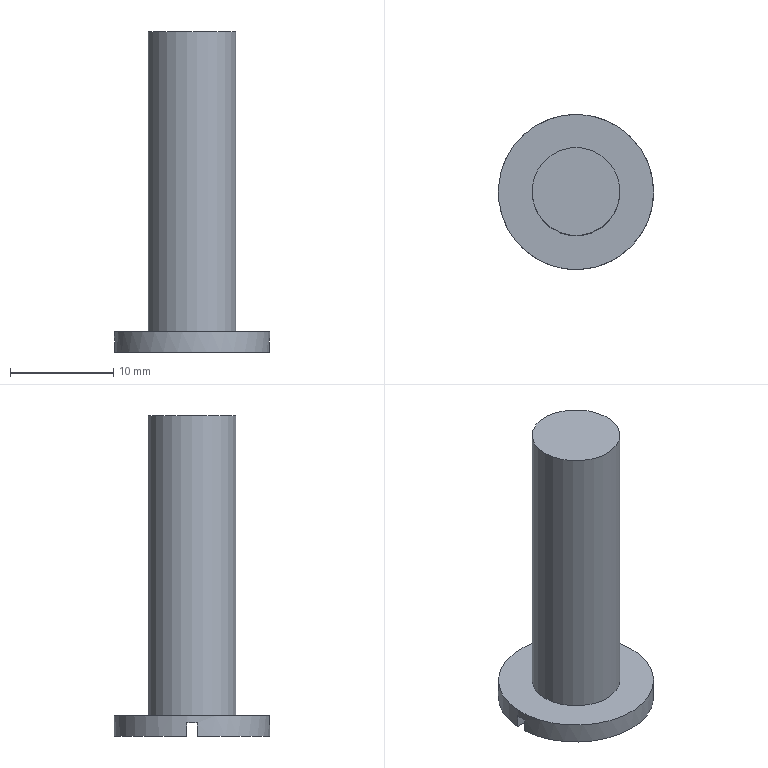Component | NX | ZYD_3 | 1 solid | 9 faces | box 15 x 15 x 31 mm | volume 1980 mm3 | plane 7 | cylinder 2 | commonest cylinder face diameters 15 x1 8.5 x1
STEP:
#1=CARTESIAN_POINT('',(0.,0.,0.));
#2=DIRECTION('',(0.,0.,1.));
#3=DIRECTION('',(1.,0.,0.));
#4=AXIS2_PLACEMENT_3D('',#1,#2,#3);
#5=CARTESIAN_POINT('',(-50.483,0.4989,325.));
#6=VERTEX_POINT('',#5);
#7=CARTESIAN_POINT('',(-35.517,0.4989,325.));
#8=VERTEX_POINT('',#7);
#9=CARTESIAN_POINT('',(-35.517,0.4989,325.));
#10=DIRECTION('',(1.,0.,0.));
#11=VECTOR('',#10,1.);
#12=LINE('',#9,#11);
#13=CARTESIAN_POINT('',(-43.,0.,325.));
#14=DIRECTION('',(0.,0.,1.));
#15=DIRECTION('',(1.,0.,0.));
#16=AXIS2_PLACEMENT_3D('',#13,#14,#15);
#17=PLANE('',#16);
#18=CARTESIAN_POINT('',(7.483,0.4989));
#19=DIRECTION('',(1.,0.));
#20=VECTOR('',#19,1.);
#21=LINE('',#18,#20);
#22=(GEOMETRIC_REPRESENTATION_CONTEXT(2)PARAMETRIC_REPRESENTATION_CONTEXT()REPRESENTATION_CONTEXT('',''));
#23=DEFINITIONAL_REPRESENTATION('',(#21),#22);
#24=PCURVE('',#17,#23);
#25=CARTESIAN_POINT('',(-35.517,0.4989,326.3));
#26=DIRECTION('',(-0.,1.,0.));
#27=DIRECTION('',(-1.,-0.,0.));
#28=AXIS2_PLACEMENT_3D('',#25,#26,#27);
#29=PLANE('',#28);
#30=CARTESIAN_POINT('',(0.,-1.3));
#31=DIRECTION('',(-1.,0.));
#32=VECTOR('',#31,1.);
#33=LINE('',#30,#32);
#34=(GEOMETRIC_REPRESENTATION_CONTEXT(2)PARAMETRIC_REPRESENTATION_CONTEXT()REPRESENTATION_CONTEXT('',''));
#35=DEFINITIONAL_REPRESENTATION('',(#33),#34);
#36=PCURVE('',#29,#35);
#37=SURFACE_CURVE('',#12,(#24,#36),.PCURVE_S1.);
#38=EDGE_CURVE('',#6,#8,#37,.T.);
#39=ORIENTED_EDGE('',*,*,#38,.F.);
#40=CARTESIAN_POINT('',(-43.,0.,325.));
#41=DIRECTION('',(0.,0.,1.));
#42=DIRECTION('',(1.,0.,0.));
#43=AXIS2_PLACEMENT_3D('',#40,#41,#42);
#44=CIRCLE('',#43,7.5);
#45=CARTESIAN_POINT('',(0.,0.));
#46=DIRECTION('',(1.,0.));
#47=AXIS2_PLACEMENT_2D('',#45,#46);
#48=CIRCLE('',#47,7.5);
#49=(GEOMETRIC_REPRESENTATION_CONTEXT(2)PARAMETRIC_REPRESENTATION_CONTEXT()REPRESENTATION_CONTEXT('',''));
#50=DEFINITIONAL_REPRESENTATION('',(#48),#49);
#51=PCURVE('',#17,#50);
#52=CARTESIAN_POINT('',(-43.,0.,327.));
#53=DIRECTION('',(0.,0.,-1.));
#54=DIRECTION('',(-1.,0.,0.));
#55=AXIS2_PLACEMENT_3D('',#52,#53,#54);
#56=CYLINDRICAL_SURFACE('',#55,7.5);
#57=CARTESIAN_POINT('',(3.142,2.));
#58=DIRECTION('',(-1.,0.));
#59=VECTOR('',#58,1.);
#60=LINE('',#57,#59);
#61=(GEOMETRIC_REPRESENTATION_CONTEXT(2)PARAMETRIC_REPRESENTATION_CONTEXT()REPRESENTATION_CONTEXT('',''));
#62=DEFINITIONAL_REPRESENTATION('',(#60),#61);
#63=PCURVE('',#56,#62);
#64=SURFACE_CURVE('',#44,(#51,#63),.PCURVE_S1.);
#65=EDGE_CURVE('',#8,#6,#64,.T.);
#66=ORIENTED_EDGE('',*,*,#65,.F.);
#67=EDGE_LOOP('',(#39,#66));
#68=FACE_BOUND('',#67,.T.);
#69=ADVANCED_FACE('',(#68),#17,.F.);
#70=CARTESIAN_POINT('',(-35.517,-0.4989,325.));
#71=VERTEX_POINT('',#70);
#72=CARTESIAN_POINT('',(-50.483,-0.4989,325.));
#73=VERTEX_POINT('',#72);
#74=CARTESIAN_POINT('',(-50.483,-0.4989,325.));
#75=DIRECTION('',(-1.,0.,0.));
#76=VECTOR('',#75,1.);
#77=LINE('',#74,#76);
#78=CARTESIAN_POINT('',(-43.,0.,325.));
#79=DIRECTION('',(0.,0.,1.));
#80=DIRECTION('',(1.,0.,0.));
#81=AXIS2_PLACEMENT_3D('',#78,#79,#80);
#82=PLANE('',#81);
#83=CARTESIAN_POINT('',(-7.483,-0.4989));
#84=DIRECTION('',(-1.,0.));
#85=VECTOR('',#84,1.);
#86=LINE('',#83,#85);
#87=(GEOMETRIC_REPRESENTATION_CONTEXT(2)PARAMETRIC_REPRESENTATION_CONTEXT()REPRESENTATION_CONTEXT('',''));
#88=DEFINITIONAL_REPRESENTATION('',(#86),#87);
#89=PCURVE('',#82,#88);
#90=CARTESIAN_POINT('',(-50.483,-0.4989,326.3));
#91=DIRECTION('',(0.,-1.,0.));
#92=DIRECTION('',(0.,0.,-1.));
#93=AXIS2_PLACEMENT_3D('',#90,#91,#92);
#94=PLANE('',#93);
#95=CARTESIAN_POINT('',(1.3,0.));
#96=DIRECTION('',(0.,-1.));
#97=VECTOR('',#96,1.);
#98=LINE('',#95,#97);
#99=(GEOMETRIC_REPRESENTATION_CONTEXT(2)PARAMETRIC_REPRESENTATION_CONTEXT()REPRESENTATION_CONTEXT('',''));
#100=DEFINITIONAL_REPRESENTATION('',(#98),#99);
#101=PCURVE('',#94,#100);
#102=SURFACE_CURVE('',#77,(#89,#101),.PCURVE_S1.);
#103=EDGE_CURVE('',#71,#73,#102,.T.);
#104=ORIENTED_EDGE('',*,*,#103,.F.);
#105=CARTESIAN_POINT('',(-43.,0.,325.));
#106=DIRECTION('',(0.,0.,1.));
#107=DIRECTION('',(1.,0.,0.));
#108=AXIS2_PLACEMENT_3D('',#105,#106,#107);
#109=CIRCLE('',#108,7.5);
#110=CARTESIAN_POINT('',(0.,0.));
#111=DIRECTION('',(1.,0.));
#112=AXIS2_PLACEMENT_2D('',#110,#111);
#113=CIRCLE('',#112,7.5);
#114=(GEOMETRIC_REPRESENTATION_CONTEXT(2)PARAMETRIC_REPRESENTATION_CONTEXT()REPRESENTATION_CONTEXT('',''));
#115=DEFINITIONAL_REPRESENTATION('',(#113),#114);
#116=PCURVE('',#82,#115);
#117=CARTESIAN_POINT('',(9.425,2.));
#118=DIRECTION('',(-1.,0.));
#119=VECTOR('',#118,1.);
#120=LINE('',#117,#119);
#121=(GEOMETRIC_REPRESENTATION_CONTEXT(2)PARAMETRIC_REPRESENTATION_CONTEXT()REPRESENTATION_CONTEXT('',''));
#122=DEFINITIONAL_REPRESENTATION('',(#120),#121);
#123=PCURVE('',#56,#122);
#124=SURFACE_CURVE('',#109,(#116,#123),.PCURVE_S1.);
#125=EDGE_CURVE('',#73,#71,#124,.T.);
#126=ORIENTED_EDGE('',*,*,#125,.F.);
#127=EDGE_LOOP('',(#104,#126));
#128=FACE_BOUND('',#127,.T.);
#129=ADVANCED_FACE('',(#128),#82,.F.);
#130=CARTESIAN_POINT('',(-35.517,0.4989,326.3));
#131=VERTEX_POINT('',#130);
#132=CARTESIAN_POINT('',(-35.517,-0.4989,326.3));
#133=VERTEX_POINT('',#132);
#134=CARTESIAN_POINT('',(-43.,0.,326.3));
#135=DIRECTION('',(0.,0.,-1.));
#136=DIRECTION('',(-1.,0.,0.));
#137=AXIS2_PLACEMENT_3D('',#134,#135,#136);
#138=CIRCLE('',#137,7.5);
#139=CARTESIAN_POINT('',(0.,0.7));
#140=DIRECTION('',(1.,0.));
#141=VECTOR('',#140,1.);
#142=LINE('',#139,#141);
#143=(GEOMETRIC_REPRESENTATION_CONTEXT(2)PARAMETRIC_REPRESENTATION_CONTEXT()REPRESENTATION_CONTEXT('',''));
#144=DEFINITIONAL_REPRESENTATION('',(#142),#143);
#145=PCURVE('',#56,#144);
#146=CARTESIAN_POINT('',(-52.183,0.4989,326.3));
#147=DIRECTION('',(0.,0.,-1.));
#148=DIRECTION('',(-1.,0.,0.));
#149=AXIS2_PLACEMENT_3D('',#146,#147,#148);
#150=PLANE('',#149);
#151=CARTESIAN_POINT('',(-9.183,-0.4989));
#152=DIRECTION('',(1.,0.));
#153=AXIS2_PLACEMENT_2D('',#151,#152);
#154=CIRCLE('',#153,7.5);
#155=(GEOMETRIC_REPRESENTATION_CONTEXT(2)PARAMETRIC_REPRESENTATION_CONTEXT()REPRESENTATION_CONTEXT('',''));
#156=DEFINITIONAL_REPRESENTATION('',(#154),#155);
#157=PCURVE('',#150,#156);
#158=SURFACE_CURVE('',#138,(#145,#157),.PCURVE_S1.);
#159=EDGE_CURVE('',#131,#133,#158,.T.);
#160=ORIENTED_EDGE('',*,*,#159,.F.);
#161=CARTESIAN_POINT('',(-35.517,0.4989,327.));
#162=DIRECTION('',(0.,0.,-1.));
#163=VECTOR('',#162,1.);
#164=LINE('',#161,#163);
#165=CARTESIAN_POINT('',(3.075,0.));
#166=DIRECTION('',(0.,1.));
#167=VECTOR('',#166,1.);
#168=LINE('',#165,#167);
#169=(GEOMETRIC_REPRESENTATION_CONTEXT(2)PARAMETRIC_REPRESENTATION_CONTEXT()REPRESENTATION_CONTEXT('',''));
#170=DEFINITIONAL_REPRESENTATION('',(#168),#169);
#171=PCURVE('',#56,#170);
#172=CARTESIAN_POINT('',(0.,0.7));
#173=DIRECTION('',(0.,-1.));
#174=VECTOR('',#173,1.);
#175=LINE('',#172,#174);
#176=(GEOMETRIC_REPRESENTATION_CONTEXT(2)PARAMETRIC_REPRESENTATION_CONTEXT()REPRESENTATION_CONTEXT('',''));
#177=DEFINITIONAL_REPRESENTATION('',(#175),#176);
#178=PCURVE('',#29,#177);
#179=SURFACE_CURVE('',#164,(#171,#178),.PCURVE_S1.);
#180=EDGE_CURVE('',#131,#8,#179,.T.);
#181=ORIENTED_EDGE('',*,*,#180,.T.);
#182=ORIENTED_EDGE('',*,*,#65,.T.);
#183=CARTESIAN_POINT('',(-50.483,0.4989,326.3));
#184=VERTEX_POINT('',#183);
#185=CARTESIAN_POINT('',(-50.483,0.4989,327.));
#186=DIRECTION('',(0.,0.,1.));
#187=VECTOR('',#186,1.);
#188=LINE('',#185,#187);
#189=CARTESIAN_POINT('',(0.06657,0.));
#190=DIRECTION('',(0.,-1.));
#191=VECTOR('',#190,1.);
#192=LINE('',#189,#191);
#193=(GEOMETRIC_REPRESENTATION_CONTEXT(2)PARAMETRIC_REPRESENTATION_CONTEXT()REPRESENTATION_CONTEXT('',''));
#194=DEFINITIONAL_REPRESENTATION('',(#192),#193);
#195=PCURVE('',#56,#194);
#196=CARTESIAN_POINT('',(14.967,0.7));
#197=DIRECTION('',(0.,1.));
#198=VECTOR('',#197,1.);
#199=LINE('',#196,#198);
#200=(GEOMETRIC_REPRESENTATION_CONTEXT(2)PARAMETRIC_REPRESENTATION_CONTEXT()REPRESENTATION_CONTEXT('',''));
#201=DEFINITIONAL_REPRESENTATION('',(#199),#200);
#202=PCURVE('',#29,#201);
#203=SURFACE_CURVE('',#188,(#195,#202),.PCURVE_S1.);
#204=EDGE_CURVE('',#6,#184,#203,.T.);
#205=ORIENTED_EDGE('',*,*,#204,.T.);
#206=CARTESIAN_POINT('',(-50.483,0.4989,327.));
#207=VERTEX_POINT('',#206);
#208=CARTESIAN_POINT('',(-50.483,0.4989,327.));
#209=CARTESIAN_POINT('',(-50.483,0.4989,326.3));
#210=B_SPLINE_CURVE_WITH_KNOTS('',1,(#208,#209),.UNSPECIFIED.,.F.,.F.,(2,2),(0.,0.7),.PIECEWISE_BEZIER_KNOTS.);
#211=CARTESIAN_POINT('',(0.06657,0.));
#212=DIRECTION('',(0.,1.));
#213=VECTOR('',#212,1.);
#214=LINE('',#211,#213);
#215=(GEOMETRIC_REPRESENTATION_CONTEXT(2)PARAMETRIC_REPRESENTATION_CONTEXT()REPRESENTATION_CONTEXT('',''));
#216=DEFINITIONAL_REPRESENTATION('',(#214),#215);
#217=PCURVE('',#56,#216);
#218=CARTESIAN_POINT('',(6.35,0.));
#219=DIRECTION('',(0.,1.));
#220=VECTOR('',#219,1.);
#221=LINE('',#218,#220);
#222=(GEOMETRIC_REPRESENTATION_CONTEXT(2)PARAMETRIC_REPRESENTATION_CONTEXT()REPRESENTATION_CONTEXT('',''));
#223=DEFINITIONAL_REPRESENTATION('',(#221),#222);
#224=PCURVE('',#56,#223);
#225=SEAM_CURVE('',#210,(#217,#224),.PCURVE_S1.);
#226=EDGE_CURVE('',#207,#184,#225,.T.);
#227=ORIENTED_EDGE('',*,*,#226,.F.);
#228=CARTESIAN_POINT('',(-35.5,0.,327.));
#229=VERTEX_POINT('',#228);
#230=CARTESIAN_POINT('',(-43.,0.,327.));
#231=DIRECTION('',(0.,0.,1.));
#232=DIRECTION('',(1.,0.,0.));
#233=AXIS2_PLACEMENT_3D('',#230,#231,#232);
#234=CIRCLE('',#233,7.5);
#235=CARTESIAN_POINT('',(3.142,0.));
#236=DIRECTION('',(-1.,0.));
#237=VECTOR('',#236,1.);
#238=LINE('',#235,#237);
#239=(GEOMETRIC_REPRESENTATION_CONTEXT(2)PARAMETRIC_REPRESENTATION_CONTEXT()REPRESENTATION_CONTEXT('',''));
#240=DEFINITIONAL_REPRESENTATION('',(#238),#239);
#241=PCURVE('',#56,#240);
#242=CARTESIAN_POINT('',(-43.,0.,327.));
#243=DIRECTION('',(0.,0.,1.));
#244=DIRECTION('',(1.,0.,0.));
#245=AXIS2_PLACEMENT_3D('',#242,#243,#244);
#246=PLANE('',#245);
#247=CARTESIAN_POINT('',(0.,0.));
#248=DIRECTION('',(1.,0.));
#249=AXIS2_PLACEMENT_2D('',#247,#248);
#250=CIRCLE('',#249,7.5);
#251=(GEOMETRIC_REPRESENTATION_CONTEXT(2)PARAMETRIC_REPRESENTATION_CONTEXT()REPRESENTATION_CONTEXT('',''));
#252=DEFINITIONAL_REPRESENTATION('',(#250),#251);
#253=PCURVE('',#246,#252);
#254=SURFACE_CURVE('',#234,(#241,#253),.PCURVE_S1.);
#255=EDGE_CURVE('',#229,#207,#254,.T.);
#256=ORIENTED_EDGE('',*,*,#255,.F.);
#257=CARTESIAN_POINT('',(-43.,0.,327.));
#258=DIRECTION('',(0.,0.,1.));
#259=DIRECTION('',(1.,0.,0.));
#260=AXIS2_PLACEMENT_3D('',#257,#258,#259);
#261=CIRCLE('',#260,7.5);
#262=CARTESIAN_POINT('',(9.425,0.));
#263=DIRECTION('',(-1.,0.));
#264=VECTOR('',#263,1.);
#265=LINE('',#262,#264);
#266=(GEOMETRIC_REPRESENTATION_CONTEXT(2)PARAMETRIC_REPRESENTATION_CONTEXT()REPRESENTATION_CONTEXT('',''));
#267=DEFINITIONAL_REPRESENTATION('',(#265),#266);
#268=PCURVE('',#56,#267);
#269=CARTESIAN_POINT('',(0.,0.));
#270=DIRECTION('',(1.,0.));
#271=AXIS2_PLACEMENT_2D('',#269,#270);
#272=CIRCLE('',#271,7.5);
#273=(GEOMETRIC_REPRESENTATION_CONTEXT(2)PARAMETRIC_REPRESENTATION_CONTEXT()REPRESENTATION_CONTEXT('',''));
#274=DEFINITIONAL_REPRESENTATION('',(#272),#273);
#275=PCURVE('',#246,#274);
#276=SURFACE_CURVE('',#261,(#268,#275),.PCURVE_S1.);
#277=EDGE_CURVE('',#207,#229,#276,.T.);
#278=ORIENTED_EDGE('',*,*,#277,.F.);
#279=ORIENTED_EDGE('',*,*,#226,.T.);
#280=CARTESIAN_POINT('',(-50.483,-0.4989,326.3));
#281=VERTEX_POINT('',#280);
#282=CARTESIAN_POINT('',(-43.,0.,326.3));
#283=DIRECTION('',(0.,0.,-1.));
#284=DIRECTION('',(-1.,0.,0.));
#285=AXIS2_PLACEMENT_3D('',#282,#283,#284);
#286=CIRCLE('',#285,7.5);
#287=CARTESIAN_POINT('',(0.,0.7));
#288=DIRECTION('',(1.,0.));
#289=VECTOR('',#288,1.);
#290=LINE('',#287,#289);
#291=(GEOMETRIC_REPRESENTATION_CONTEXT(2)PARAMETRIC_REPRESENTATION_CONTEXT()REPRESENTATION_CONTEXT('',''));
#292=DEFINITIONAL_REPRESENTATION('',(#290),#291);
#293=PCURVE('',#56,#292);
#294=CARTESIAN_POINT('',(-9.183,-0.4989));
#295=DIRECTION('',(1.,0.));
#296=AXIS2_PLACEMENT_2D('',#294,#295);
#297=CIRCLE('',#296,7.5);
#298=(GEOMETRIC_REPRESENTATION_CONTEXT(2)PARAMETRIC_REPRESENTATION_CONTEXT()REPRESENTATION_CONTEXT('',''));
#299=DEFINITIONAL_REPRESENTATION('',(#297),#298);
#300=PCURVE('',#150,#299);
#301=SURFACE_CURVE('',#286,(#293,#300),.PCURVE_S1.);
#302=EDGE_CURVE('',#281,#184,#301,.T.);
#303=ORIENTED_EDGE('',*,*,#302,.F.);
#304=CARTESIAN_POINT('',(-50.483,-0.4989,327.));
#305=DIRECTION('',(0.,0.,-1.));
#306=VECTOR('',#305,1.);
#307=LINE('',#304,#306);
#308=CARTESIAN_POINT('',(6.217,0.));
#309=DIRECTION('',(0.,1.));
#310=VECTOR('',#309,1.);
#311=LINE('',#308,#310);
#312=(GEOMETRIC_REPRESENTATION_CONTEXT(2)PARAMETRIC_REPRESENTATION_CONTEXT()REPRESENTATION_CONTEXT('',''));
#313=DEFINITIONAL_REPRESENTATION('',(#311),#312);
#314=PCURVE('',#56,#313);
#315=CARTESIAN_POINT('',(-0.7,0.));
#316=DIRECTION('',(1.,0.));
#317=VECTOR('',#316,1.);
#318=LINE('',#315,#317);
#319=(GEOMETRIC_REPRESENTATION_CONTEXT(2)PARAMETRIC_REPRESENTATION_CONTEXT()REPRESENTATION_CONTEXT('',''));
#320=DEFINITIONAL_REPRESENTATION('',(#318),#319);
#321=PCURVE('',#94,#320);
#322=SURFACE_CURVE('',#307,(#314,#321),.PCURVE_S1.);
#323=EDGE_CURVE('',#281,#73,#322,.T.);
#324=ORIENTED_EDGE('',*,*,#323,.T.);
#325=ORIENTED_EDGE('',*,*,#125,.T.);
#326=CARTESIAN_POINT('',(-35.517,-0.4989,327.));
#327=DIRECTION('',(0.,0.,1.));
#328=VECTOR('',#327,1.);
#329=LINE('',#326,#328);
#330=CARTESIAN_POINT('',(3.208,0.));
#331=DIRECTION('',(0.,-1.));
#332=VECTOR('',#331,1.);
#333=LINE('',#330,#332);
#334=(GEOMETRIC_REPRESENTATION_CONTEXT(2)PARAMETRIC_REPRESENTATION_CONTEXT()REPRESENTATION_CONTEXT('',''));
#335=DEFINITIONAL_REPRESENTATION('',(#333),#334);
#336=PCURVE('',#56,#335);
#337=CARTESIAN_POINT('',(-0.7,14.967));
#338=DIRECTION('',(-1.,0.));
#339=VECTOR('',#338,1.);
#340=LINE('',#337,#339);
#341=(GEOMETRIC_REPRESENTATION_CONTEXT(2)PARAMETRIC_REPRESENTATION_CONTEXT()REPRESENTATION_CONTEXT('',''));
#342=DEFINITIONAL_REPRESENTATION('',(#340),#341);
#343=PCURVE('',#94,#342);
#344=SURFACE_CURVE('',#329,(#336,#343),.PCURVE_S1.);
#345=EDGE_CURVE('',#71,#133,#344,.T.);
#346=ORIENTED_EDGE('',*,*,#345,.T.);
#347=EDGE_LOOP('',(#160,#181,#182,#205,#227,#256,#278,#279,#303,#324,#325,#346));
#348=FACE_BOUND('',#347,.T.);
#349=ADVANCED_FACE('',(#348),#56,.T.);
#350=CARTESIAN_POINT('',(-38.75,0.,327.));
#351=VERTEX_POINT('',#350);
#352=CARTESIAN_POINT('',(-43.,0.,327.));
#353=DIRECTION('',(0.,0.,1.));
#354=DIRECTION('',(1.,0.,0.));
#355=AXIS2_PLACEMENT_3D('',#352,#353,#354);
#356=CIRCLE('',#355,4.25);
#357=CARTESIAN_POINT('',(0.,0.));
#358=DIRECTION('',(1.,0.));
#359=AXIS2_PLACEMENT_2D('',#357,#358);
#360=CIRCLE('',#359,4.25);
#361=(GEOMETRIC_REPRESENTATION_CONTEXT(2)PARAMETRIC_REPRESENTATION_CONTEXT()REPRESENTATION_CONTEXT('',''));
#362=DEFINITIONAL_REPRESENTATION('',(#360),#361);
#363=PCURVE('',#246,#362);
#364=CARTESIAN_POINT('',(-43.,0.,356.));
#365=DIRECTION('',(0.,0.,-1.));
#366=DIRECTION('',(-1.,0.,0.));
#367=AXIS2_PLACEMENT_3D('',#364,#365,#366);
#368=CYLINDRICAL_SURFACE('',#367,4.25);
#369=CARTESIAN_POINT('',(9.425,29.));
#370=DIRECTION('',(-1.,0.));
#371=VECTOR('',#370,1.);
#372=LINE('',#369,#371);
#373=(GEOMETRIC_REPRESENTATION_CONTEXT(2)PARAMETRIC_REPRESENTATION_CONTEXT()REPRESENTATION_CONTEXT('',''));
#374=DEFINITIONAL_REPRESENTATION('',(#372),#373);
#375=PCURVE('',#368,#374);
#376=SURFACE_CURVE('',#356,(#363,#375),.PCURVE_S1.);
#377=EDGE_CURVE('',#351,#351,#376,.T.);
#378=ORIENTED_EDGE('',*,*,#377,.F.);
#379=EDGE_LOOP('',(#378));
#380=FACE_BOUND('',#379,.T.);
#381=ORIENTED_EDGE('',*,*,#255,.T.);
#382=ORIENTED_EDGE('',*,*,#277,.T.);
#383=EDGE_LOOP('',(#381,#382));
#384=FACE_BOUND('',#383,.T.);
#385=ADVANCED_FACE('',(#380,#384),#246,.T.);
#386=CARTESIAN_POINT('',(-38.75,0.,356.));
#387=VERTEX_POINT('',#386);
#388=CARTESIAN_POINT('',(-43.,0.,356.));
#389=DIRECTION('',(0.,0.,1.));
#390=DIRECTION('',(1.,0.,0.));
#391=AXIS2_PLACEMENT_3D('',#388,#389,#390);
#392=CIRCLE('',#391,4.25);
#393=CARTESIAN_POINT('',(9.425,0.));
#394=DIRECTION('',(-1.,0.));
#395=VECTOR('',#394,1.);
#396=LINE('',#393,#395);
#397=(GEOMETRIC_REPRESENTATION_CONTEXT(2)PARAMETRIC_REPRESENTATION_CONTEXT()REPRESENTATION_CONTEXT('',''));
#398=DEFINITIONAL_REPRESENTATION('',(#396),#397);
#399=PCURVE('',#368,#398);
#400=CARTESIAN_POINT('',(-43.,0.,356.));
#401=DIRECTION('',(0.,0.,1.));
#402=DIRECTION('',(1.,0.,0.));
#403=AXIS2_PLACEMENT_3D('',#400,#401,#402);
#404=PLANE('',#403);
#405=CARTESIAN_POINT('',(0.,0.));
#406=DIRECTION('',(1.,0.));
#407=AXIS2_PLACEMENT_2D('',#405,#406);
#408=CIRCLE('',#407,4.25);
#409=(GEOMETRIC_REPRESENTATION_CONTEXT(2)PARAMETRIC_REPRESENTATION_CONTEXT()REPRESENTATION_CONTEXT('',''));
#410=DEFINITIONAL_REPRESENTATION('',(#408),#409);
#411=PCURVE('',#404,#410);
#412=SURFACE_CURVE('',#392,(#399,#411),.PCURVE_S1.);
#413=EDGE_CURVE('',#387,#387,#412,.T.);
#414=ORIENTED_EDGE('',*,*,#413,.F.);
#415=CARTESIAN_POINT('',(-38.75,0.,356.));
#416=CARTESIAN_POINT('',(-38.75,0.,327.));
#417=B_SPLINE_CURVE_WITH_KNOTS('',1,(#415,#416),.UNSPECIFIED.,.F.,.F.,(2,2),(0.,29.),.PIECEWISE_BEZIER_KNOTS.);
#418=CARTESIAN_POINT('',(9.425,0.));
#419=DIRECTION('',(0.,1.));
#420=VECTOR('',#419,1.);
#421=LINE('',#418,#420);
#422=(GEOMETRIC_REPRESENTATION_CONTEXT(2)PARAMETRIC_REPRESENTATION_CONTEXT()REPRESENTATION_CONTEXT('',''));
#423=DEFINITIONAL_REPRESENTATION('',(#421),#422);
#424=PCURVE('',#368,#423);
#425=CARTESIAN_POINT('',(3.142,0.));
#426=DIRECTION('',(0.,1.));
#427=VECTOR('',#426,1.);
#428=LINE('',#425,#427);
#429=(GEOMETRIC_REPRESENTATION_CONTEXT(2)PARAMETRIC_REPRESENTATION_CONTEXT()REPRESENTATION_CONTEXT('',''));
#430=DEFINITIONAL_REPRESENTATION('',(#428),#429);
#431=PCURVE('',#368,#430);
#432=SEAM_CURVE('',#417,(#424,#431),.PCURVE_S1.);
#433=EDGE_CURVE('',#387,#351,#432,.T.);
#434=ORIENTED_EDGE('',*,*,#433,.T.);
#435=ORIENTED_EDGE('',*,*,#377,.T.);
#436=ORIENTED_EDGE('',*,*,#433,.F.);
#437=EDGE_LOOP('',(#414,#434,#435,#436));
#438=FACE_BOUND('',#437,.T.);
#439=ADVANCED_FACE('',(#438),#368,.T.);
#440=ORIENTED_EDGE('',*,*,#413,.T.);
#441=EDGE_LOOP('',(#440));
#442=FACE_BOUND('',#441,.T.);
#443=ADVANCED_FACE('',(#442),#404,.T.);
#444=ORIENTED_EDGE('',*,*,#159,.T.);
#445=CARTESIAN_POINT('',(-33.809,-0.4989,326.3));
#446=DIRECTION('',(-1.,-0.,0.));
#447=VECTOR('',#446,1.);
#448=LINE('',#445,#447);
#449=CARTESIAN_POINT('',(-18.375,-0.9978));
#450=DIRECTION('',(1.,-0.));
#451=VECTOR('',#450,1.);
#452=LINE('',#449,#451);
#453=(GEOMETRIC_REPRESENTATION_CONTEXT(2)PARAMETRIC_REPRESENTATION_CONTEXT()REPRESENTATION_CONTEXT('',''));
#454=DEFINITIONAL_REPRESENTATION('',(#452),#453);
#455=PCURVE('',#150,#454);
#456=CARTESIAN_POINT('',(0.,16.675));
#457=DIRECTION('',(0.,-1.));
#458=VECTOR('',#457,1.);
#459=LINE('',#456,#458);
#460=(GEOMETRIC_REPRESENTATION_CONTEXT(2)PARAMETRIC_REPRESENTATION_CONTEXT()REPRESENTATION_CONTEXT('',''));
#461=DEFINITIONAL_REPRESENTATION('',(#459),#460);
#462=PCURVE('',#94,#461);
#463=SURFACE_CURVE('',#448,(#455,#462),.PCURVE_S1.);
#464=EDGE_CURVE('',#133,#281,#463,.T.);
#465=ORIENTED_EDGE('',*,*,#464,.T.);
#466=ORIENTED_EDGE('',*,*,#302,.T.);
#467=CARTESIAN_POINT('',(-52.183,0.4989,326.3));
#468=DIRECTION('',(1.,0.,0.));
#469=VECTOR('',#468,1.);
#470=LINE('',#467,#469);
#471=CARTESIAN_POINT('',(0.,0.));
#472=DIRECTION('',(-1.,0.));
#473=VECTOR('',#472,1.);
#474=LINE('',#471,#473);
#475=(GEOMETRIC_REPRESENTATION_CONTEXT(2)PARAMETRIC_REPRESENTATION_CONTEXT()REPRESENTATION_CONTEXT('',''));
#476=DEFINITIONAL_REPRESENTATION('',(#474),#475);
#477=PCURVE('',#150,#476);
#478=CARTESIAN_POINT('',(16.667,0.));
#479=DIRECTION('',(-1.,0.));
#480=VECTOR('',#479,1.);
#481=LINE('',#478,#480);
#482=(GEOMETRIC_REPRESENTATION_CONTEXT(2)PARAMETRIC_REPRESENTATION_CONTEXT()REPRESENTATION_CONTEXT('',''));
#483=DEFINITIONAL_REPRESENTATION('',(#481),#482);
#484=PCURVE('',#29,#483);
#485=SURFACE_CURVE('',#470,(#477,#484),.PCURVE_S1.);
#486=EDGE_CURVE('',#184,#131,#485,.T.);
#487=ORIENTED_EDGE('',*,*,#486,.T.);
#488=EDGE_LOOP('',(#444,#465,#466,#487));
#489=FACE_BOUND('',#488,.T.);
#490=ADVANCED_FACE('',(#489),#150,.T.);
#491=ORIENTED_EDGE('',*,*,#486,.F.);
#492=ORIENTED_EDGE('',*,*,#204,.F.);
#493=ORIENTED_EDGE('',*,*,#38,.T.);
#494=ORIENTED_EDGE('',*,*,#180,.F.);
#495=EDGE_LOOP('',(#491,#492,#493,#494));
#496=FACE_BOUND('',#495,.T.);
#497=ADVANCED_FACE('',(#496),#29,.F.);
#498=ORIENTED_EDGE('',*,*,#464,.F.);
#499=ORIENTED_EDGE('',*,*,#345,.F.);
#500=ORIENTED_EDGE('',*,*,#103,.T.);
#501=ORIENTED_EDGE('',*,*,#323,.F.);
#502=EDGE_LOOP('',(#498,#499,#500,#501));
#503=FACE_BOUND('',#502,.T.);
#504=ADVANCED_FACE('',(#503),#94,.F.);
#505=CLOSED_SHELL('',(#69,#129,#349,#385,#439,#443,#490,#497,#504));
#506=MANIFOLD_SOLID_BREP('',#505);
#507=(LENGTH_UNIT()NAMED_UNIT(*)SI_UNIT(.MILLI.,.METRE.));
#508=UNCERTAINTY_MEASURE_WITH_UNIT(LENGTH_MEASURE(0.000002),#507,'','');
#509=(NAMED_UNIT(*)PLANE_ANGLE_UNIT()SI_UNIT($,.RADIAN.));
#510=(NAMED_UNIT(*)SI_UNIT($,.STERADIAN.)SOLID_ANGLE_UNIT());
#511=(GEOMETRIC_REPRESENTATION_CONTEXT(3)GLOBAL_UNCERTAINTY_ASSIGNED_CONTEXT((#508))GLOBAL_UNIT_ASSIGNED_CONTEXT((#507,#509,#510))REPRESENTATION_CONTEXT('',''));
#512=ADVANCED_BREP_SHAPE_REPRESENTATION('',(#4,#506),#511);